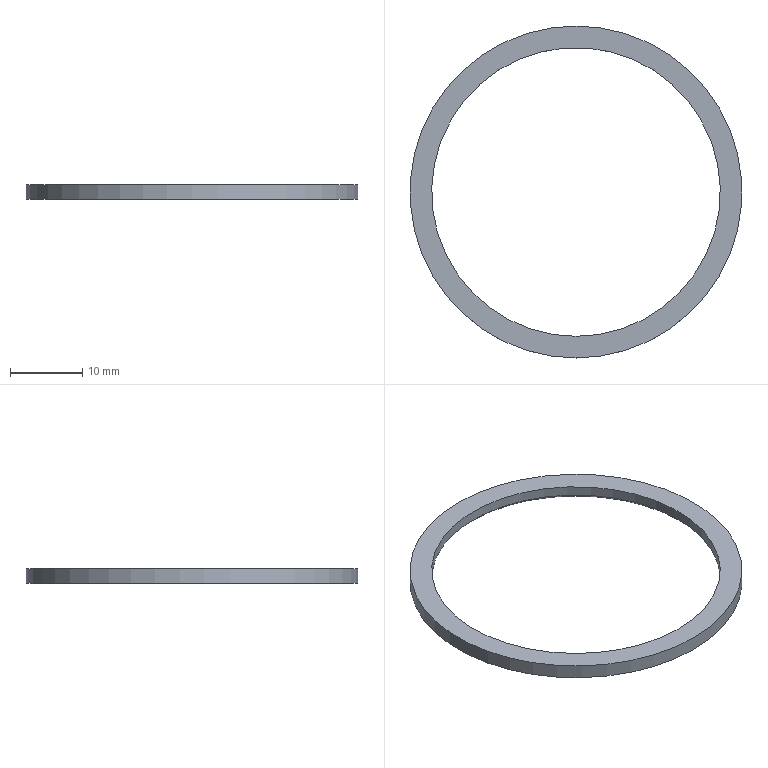Component | NX | END_CAP_SEAL | 1 solid | 5 faces | box 46 x 46 x 2 mm | volume 788 mm3 | cylinder 2 | plane 2 | cone 1 | commonest cylinder face diameters 46 x1 40 x1
STEP:
#1=CARTESIAN_POINT('',(0.,0.,0.));
#2=DIRECTION('',(0.,0.,1.));
#3=DIRECTION('',(1.,0.,0.));
#4=AXIS2_PLACEMENT_3D('',#1,#2,#3);
#5=CARTESIAN_POINT('',(0.,-23.,-137.));
#6=VERTEX_POINT('',#5);
#7=CARTESIAN_POINT('',(0.,-0.,-137.));
#8=DIRECTION('',(0.,0.,1.));
#9=DIRECTION('',(0.,-1.,0.));
#10=AXIS2_PLACEMENT_3D('',#7,#8,#9);
#11=CIRCLE('',#10,23.);
#12=CARTESIAN_POINT('',(0.,-0.,-137.));
#13=DIRECTION('',(0.,0.,-1.));
#14=DIRECTION('',(0.,1.,0.));
#15=AXIS2_PLACEMENT_3D('',#12,#13,#14);
#16=CYLINDRICAL_SURFACE('',#15,23.);
#17=CARTESIAN_POINT('',(9.425,0.));
#18=DIRECTION('',(-1.,0.));
#19=VECTOR('',#18,1.);
#20=LINE('',#17,#19);
#21=(GEOMETRIC_REPRESENTATION_CONTEXT(2)PARAMETRIC_REPRESENTATION_CONTEXT()REPRESENTATION_CONTEXT('',''));
#22=DEFINITIONAL_REPRESENTATION('',(#20),#21);
#23=PCURVE('',#16,#22);
#24=CARTESIAN_POINT('',(0.,-0.,-137.));
#25=DIRECTION('',(0.,0.,1.));
#26=DIRECTION('',(0.,-1.,0.));
#27=AXIS2_PLACEMENT_3D('',#24,#25,#26);
#28=PLANE('',#27);
#29=CARTESIAN_POINT('',(0.,0.));
#30=DIRECTION('',(1.,0.));
#31=AXIS2_PLACEMENT_2D('',#29,#30);
#32=CIRCLE('',#31,23.);
#33=(GEOMETRIC_REPRESENTATION_CONTEXT(2)PARAMETRIC_REPRESENTATION_CONTEXT()REPRESENTATION_CONTEXT('',''));
#34=DEFINITIONAL_REPRESENTATION('',(#32),#33);
#35=PCURVE('',#28,#34);
#36=SURFACE_CURVE('',#11,(#23,#35),.PCURVE_S1.);
#37=EDGE_CURVE('',#6,#6,#36,.T.);
#38=ORIENTED_EDGE('',*,*,#37,.F.);
#39=CARTESIAN_POINT('',(0.,-23.,-139.));
#40=VERTEX_POINT('',#39);
#41=CARTESIAN_POINT('',(0.,-23.,-137.));
#42=CARTESIAN_POINT('',(0.,-23.,-139.));
#43=B_SPLINE_CURVE_WITH_KNOTS('',1,(#41,#42),.UNSPECIFIED.,.F.,.F.,(2,2),(0.,2.),.PIECEWISE_BEZIER_KNOTS.);
#44=CARTESIAN_POINT('',(9.425,0.));
#45=DIRECTION('',(0.,1.));
#46=VECTOR('',#45,1.);
#47=LINE('',#44,#46);
#48=(GEOMETRIC_REPRESENTATION_CONTEXT(2)PARAMETRIC_REPRESENTATION_CONTEXT()REPRESENTATION_CONTEXT('',''));
#49=DEFINITIONAL_REPRESENTATION('',(#47),#48);
#50=PCURVE('',#16,#49);
#51=CARTESIAN_POINT('',(3.142,0.));
#52=DIRECTION('',(0.,1.));
#53=VECTOR('',#52,1.);
#54=LINE('',#51,#53);
#55=(GEOMETRIC_REPRESENTATION_CONTEXT(2)PARAMETRIC_REPRESENTATION_CONTEXT()REPRESENTATION_CONTEXT('',''));
#56=DEFINITIONAL_REPRESENTATION('',(#54),#55);
#57=PCURVE('',#16,#56);
#58=SEAM_CURVE('',#43,(#50,#57),.PCURVE_S1.);
#59=EDGE_CURVE('',#6,#40,#58,.T.);
#60=ORIENTED_EDGE('',*,*,#59,.T.);
#61=CARTESIAN_POINT('',(0.,-0.,-139.));
#62=DIRECTION('',(0.,0.,1.));
#63=DIRECTION('',(0.,-1.,0.));
#64=AXIS2_PLACEMENT_3D('',#61,#62,#63);
#65=CIRCLE('',#64,23.);
#66=CARTESIAN_POINT('',(9.425,2.));
#67=DIRECTION('',(-1.,0.));
#68=VECTOR('',#67,1.);
#69=LINE('',#66,#68);
#70=(GEOMETRIC_REPRESENTATION_CONTEXT(2)PARAMETRIC_REPRESENTATION_CONTEXT()REPRESENTATION_CONTEXT('',''));
#71=DEFINITIONAL_REPRESENTATION('',(#69),#70);
#72=PCURVE('',#16,#71);
#73=CARTESIAN_POINT('',(0.,-0.,-139.));
#74=DIRECTION('',(0.,0.,1.));
#75=DIRECTION('',(0.,-1.,0.));
#76=AXIS2_PLACEMENT_3D('',#73,#74,#75);
#77=PLANE('',#76);
#78=CARTESIAN_POINT('',(0.,0.));
#79=DIRECTION('',(1.,0.));
#80=AXIS2_PLACEMENT_2D('',#78,#79);
#81=CIRCLE('',#80,23.);
#82=(GEOMETRIC_REPRESENTATION_CONTEXT(2)PARAMETRIC_REPRESENTATION_CONTEXT()REPRESENTATION_CONTEXT('',''));
#83=DEFINITIONAL_REPRESENTATION('',(#81),#82);
#84=PCURVE('',#77,#83);
#85=SURFACE_CURVE('',#65,(#72,#84),.PCURVE_S1.);
#86=EDGE_CURVE('',#40,#40,#85,.T.);
#87=ORIENTED_EDGE('',*,*,#86,.T.);
#88=ORIENTED_EDGE('',*,*,#59,.F.);
#89=EDGE_LOOP('',(#38,#60,#87,#88));
#90=FACE_BOUND('',#89,.T.);
#91=ADVANCED_FACE('',(#90),#16,.T.);
#92=CARTESIAN_POINT('',(0.,-20.,-138.4));
#93=VERTEX_POINT('',#92);
#94=CARTESIAN_POINT('',(0.,-0.,-138.4));
#95=DIRECTION('',(0.,0.,-1.));
#96=DIRECTION('',(0.,-1.,0.));
#97=AXIS2_PLACEMENT_3D('',#94,#95,#96);
#98=CIRCLE('',#97,20.);
#99=CARTESIAN_POINT('',(0.,-0.,-137.));
#100=DIRECTION('',(0.,0.,-1.));
#101=DIRECTION('',(0.,1.,0.));
#102=AXIS2_PLACEMENT_3D('',#99,#100,#101);
#103=CYLINDRICAL_SURFACE('',#102,20.);
#104=CARTESIAN_POINT('',(3.142,1.4));
#105=DIRECTION('',(1.,0.));
#106=VECTOR('',#105,1.);
#107=LINE('',#104,#106);
#108=(GEOMETRIC_REPRESENTATION_CONTEXT(2)PARAMETRIC_REPRESENTATION_CONTEXT()REPRESENTATION_CONTEXT('',''));
#109=DEFINITIONAL_REPRESENTATION('',(#107),#108);
#110=PCURVE('',#103,#109);
#111=CARTESIAN_POINT('',(0.,-0.,-139.));
#112=DIRECTION('',(0.,0.,-1.));
#113=DIRECTION('',(0.,1.,0.));
#114=AXIS2_PLACEMENT_3D('',#111,#112,#113);
#115=CONICAL_SURFACE('',#114,20.6,0.7854);
#116=CARTESIAN_POINT('',(3.142,-0.6));
#117=DIRECTION('',(1.,0.));
#118=VECTOR('',#117,1.);
#119=LINE('',#116,#118);
#120=(GEOMETRIC_REPRESENTATION_CONTEXT(2)PARAMETRIC_REPRESENTATION_CONTEXT()REPRESENTATION_CONTEXT('',''));
#121=DEFINITIONAL_REPRESENTATION('',(#119),#120);
#122=PCURVE('',#115,#121);
#123=SURFACE_CURVE('',#98,(#110,#122),.PCURVE_S1.);
#124=EDGE_CURVE('',#93,#93,#123,.T.);
#125=ORIENTED_EDGE('',*,*,#124,.F.);
#126=CARTESIAN_POINT('',(0.,-20.,-137.));
#127=VERTEX_POINT('',#126);
#128=CARTESIAN_POINT('',(0.,-20.,-137.));
#129=CARTESIAN_POINT('',(0.,-20.,-138.4));
#130=B_SPLINE_CURVE_WITH_KNOTS('',1,(#128,#129),.UNSPECIFIED.,.F.,.F.,(2,2),(0.,1.4),.PIECEWISE_BEZIER_KNOTS.);
#131=CARTESIAN_POINT('',(3.142,0.));
#132=DIRECTION('',(0.,1.));
#133=VECTOR('',#132,1.);
#134=LINE('',#131,#133);
#135=(GEOMETRIC_REPRESENTATION_CONTEXT(2)PARAMETRIC_REPRESENTATION_CONTEXT()REPRESENTATION_CONTEXT('',''));
#136=DEFINITIONAL_REPRESENTATION('',(#134),#135);
#137=PCURVE('',#103,#136);
#138=CARTESIAN_POINT('',(9.425,0.));
#139=DIRECTION('',(0.,1.));
#140=VECTOR('',#139,1.);
#141=LINE('',#138,#140);
#142=(GEOMETRIC_REPRESENTATION_CONTEXT(2)PARAMETRIC_REPRESENTATION_CONTEXT()REPRESENTATION_CONTEXT('',''));
#143=DEFINITIONAL_REPRESENTATION('',(#141),#142);
#144=PCURVE('',#103,#143);
#145=SEAM_CURVE('',#130,(#137,#144),.PCURVE_S1.);
#146=EDGE_CURVE('',#127,#93,#145,.T.);
#147=ORIENTED_EDGE('',*,*,#146,.F.);
#148=CARTESIAN_POINT('',(0.,-0.,-137.));
#149=DIRECTION('',(0.,0.,1.));
#150=DIRECTION('',(0.,-1.,0.));
#151=AXIS2_PLACEMENT_3D('',#148,#149,#150);
#152=CIRCLE('',#151,20.);
#153=CARTESIAN_POINT('',(9.425,0.));
#154=DIRECTION('',(-1.,0.));
#155=VECTOR('',#154,1.);
#156=LINE('',#153,#155);
#157=(GEOMETRIC_REPRESENTATION_CONTEXT(2)PARAMETRIC_REPRESENTATION_CONTEXT()REPRESENTATION_CONTEXT('',''));
#158=DEFINITIONAL_REPRESENTATION('',(#156),#157);
#159=PCURVE('',#103,#158);
#160=CARTESIAN_POINT('',(0.,0.));
#161=DIRECTION('',(1.,0.));
#162=AXIS2_PLACEMENT_2D('',#160,#161);
#163=CIRCLE('',#162,20.);
#164=(GEOMETRIC_REPRESENTATION_CONTEXT(2)PARAMETRIC_REPRESENTATION_CONTEXT()REPRESENTATION_CONTEXT('',''));
#165=DEFINITIONAL_REPRESENTATION('',(#163),#164);
#166=PCURVE('',#28,#165);
#167=SURFACE_CURVE('',#152,(#159,#166),.PCURVE_S1.);
#168=EDGE_CURVE('',#127,#127,#167,.T.);
#169=ORIENTED_EDGE('',*,*,#168,.F.);
#170=ORIENTED_EDGE('',*,*,#146,.T.);
#171=EDGE_LOOP('',(#125,#147,#169,#170));
#172=FACE_BOUND('',#171,.F.);
#173=ADVANCED_FACE('',(#172),#103,.F.);
#174=ORIENTED_EDGE('',*,*,#37,.T.);
#175=EDGE_LOOP('',(#174));
#176=FACE_BOUND('',#175,.T.);
#177=ORIENTED_EDGE('',*,*,#168,.F.);
#178=EDGE_LOOP('',(#177));
#179=FACE_BOUND('',#178,.T.);
#180=ADVANCED_FACE('',(#176,#179),#28,.T.);
#181=CARTESIAN_POINT('',(0.,-20.6,-139.));
#182=VERTEX_POINT('',#181);
#183=CARTESIAN_POINT('',(0.,-0.,-139.));
#184=DIRECTION('',(0.,0.,1.));
#185=DIRECTION('',(0.,-1.,0.));
#186=AXIS2_PLACEMENT_3D('',#183,#184,#185);
#187=CIRCLE('',#186,20.6);
#188=CARTESIAN_POINT('',(0.,0.));
#189=DIRECTION('',(1.,0.));
#190=AXIS2_PLACEMENT_2D('',#188,#189);
#191=CIRCLE('',#190,20.6);
#192=(GEOMETRIC_REPRESENTATION_CONTEXT(2)PARAMETRIC_REPRESENTATION_CONTEXT()REPRESENTATION_CONTEXT('',''));
#193=DEFINITIONAL_REPRESENTATION('',(#191),#192);
#194=PCURVE('',#77,#193);
#195=CARTESIAN_POINT('',(9.425,0.));
#196=DIRECTION('',(-1.,0.));
#197=VECTOR('',#196,1.);
#198=LINE('',#195,#197);
#199=(GEOMETRIC_REPRESENTATION_CONTEXT(2)PARAMETRIC_REPRESENTATION_CONTEXT()REPRESENTATION_CONTEXT('',''));
#200=DEFINITIONAL_REPRESENTATION('',(#198),#199);
#201=PCURVE('',#115,#200);
#202=SURFACE_CURVE('',#187,(#194,#201),.PCURVE_S1.);
#203=EDGE_CURVE('',#182,#182,#202,.T.);
#204=ORIENTED_EDGE('',*,*,#203,.T.);
#205=EDGE_LOOP('',(#204));
#206=FACE_BOUND('',#205,.T.);
#207=ORIENTED_EDGE('',*,*,#86,.F.);
#208=EDGE_LOOP('',(#207));
#209=FACE_BOUND('',#208,.T.);
#210=ADVANCED_FACE('',(#206,#209),#77,.F.);
#211=ORIENTED_EDGE('',*,*,#124,.T.);
#212=CARTESIAN_POINT('',(0.,-20.,-138.4));
#213=CARTESIAN_POINT('',(0.,-20.6,-139.));
#214=B_SPLINE_CURVE_WITH_KNOTS('',1,(#212,#213),.UNSPECIFIED.,.F.,.F.,(2,2),(-0.8485,0.),.PIECEWISE_BEZIER_KNOTS.);
#215=CARTESIAN_POINT('',(9.425,0.));
#216=DIRECTION('',(0.,1.));
#217=VECTOR('',#216,1.);
#218=LINE('',#215,#217);
#219=(GEOMETRIC_REPRESENTATION_CONTEXT(2)PARAMETRIC_REPRESENTATION_CONTEXT()REPRESENTATION_CONTEXT('',''));
#220=DEFINITIONAL_REPRESENTATION('',(#218),#219);
#221=PCURVE('',#115,#220);
#222=CARTESIAN_POINT('',(3.142,0.));
#223=DIRECTION('',(0.,1.));
#224=VECTOR('',#223,1.);
#225=LINE('',#222,#224);
#226=(GEOMETRIC_REPRESENTATION_CONTEXT(2)PARAMETRIC_REPRESENTATION_CONTEXT()REPRESENTATION_CONTEXT('',''));
#227=DEFINITIONAL_REPRESENTATION('',(#225),#226);
#228=PCURVE('',#115,#227);
#229=SEAM_CURVE('',#214,(#221,#228),.PCURVE_S1.);
#230=EDGE_CURVE('',#93,#182,#229,.T.);
#231=ORIENTED_EDGE('',*,*,#230,.T.);
#232=ORIENTED_EDGE('',*,*,#203,.T.);
#233=ORIENTED_EDGE('',*,*,#230,.F.);
#234=EDGE_LOOP('',(#211,#231,#232,#233));
#235=FACE_BOUND('',#234,.F.);
#236=ADVANCED_FACE('',(#235),#115,.F.);
#237=CLOSED_SHELL('',(#91,#173,#180,#210,#236));
#238=MANIFOLD_SOLID_BREP('',#237);
#239=(LENGTH_UNIT()NAMED_UNIT(*)SI_UNIT(.MILLI.,.METRE.));
#240=UNCERTAINTY_MEASURE_WITH_UNIT(LENGTH_MEASURE(0.00001),#239,'','');
#241=(NAMED_UNIT(*)PLANE_ANGLE_UNIT()SI_UNIT($,.RADIAN.));
#242=(NAMED_UNIT(*)SI_UNIT($,.STERADIAN.)SOLID_ANGLE_UNIT());
#243=(GEOMETRIC_REPRESENTATION_CONTEXT(3)GLOBAL_UNCERTAINTY_ASSIGNED_CONTEXT((#240))GLOBAL_UNIT_ASSIGNED_CONTEXT((#239,#241,#242))REPRESENTATION_CONTEXT('',''));
#244=ADVANCED_BREP_SHAPE_REPRESENTATION('',(#4,#238),#243);